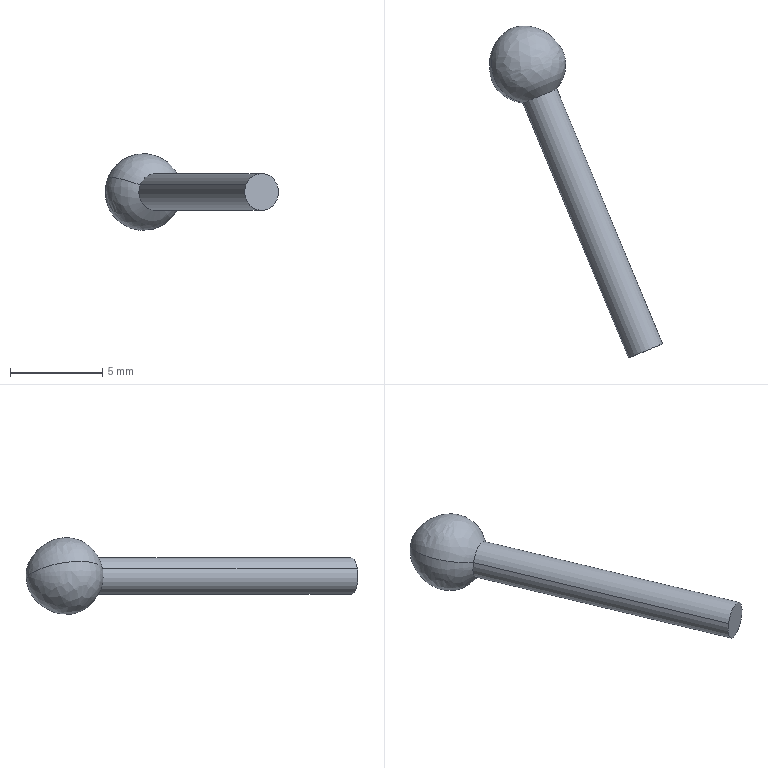Component | SolidWorks | FixedSign-2 | 1 solid | 5 faces | box 9.42 x 18.04 x 4.17 mm | volume 85 mm3 | spline 2 | cylinder 2 | plane 1 | commonest cylinder face diameters 2 x2
STEP:
#1=COLOUR_RGB('',0.7922,0.8196,0.9333);
#2=FILL_AREA_STYLE_COLOUR('',#1);
#3=FILL_AREA_STYLE('',(#2));
#4=SURFACE_STYLE_FILL_AREA(#3);
#5=SURFACE_SIDE_STYLE('',(#4));
#6=SURFACE_STYLE_USAGE(.BOTH.,#5);
#7=PRESENTATION_STYLE_ASSIGNMENT((#6));
#8=CARTESIAN_POINT('',(1.156,0.4229,15.565));
#9=VERTEX_POINT('',#8);
#10=CARTESIAN_POINT('',(1.182,0.264,15.58));
#11=VERTEX_POINT('',#10);
#12=CARTESIAN_POINT('',(1.156,0.4229,15.565));
#13=CARTESIAN_POINT('',(1.095,0.3958,15.592));
#14=CARTESIAN_POINT('',(1.093,0.2788,15.612));
#15=CARTESIAN_POINT('',(1.182,0.264,15.58));
#16=B_SPLINE_CURVE_WITH_KNOTS('',3,(#12,#13,#14,#15),.UNSPECIFIED.,.F.,.F.,(4,4),(0.,1.),.UNSPECIFIED.);
#17=EDGE_CURVE('',#9,#11,#16,.T.);
#18=ORIENTED_EDGE('',*,*,#17,.F.);
#19=CARTESIAN_POINT('',(1.249,0.2919,15.55));
#20=VERTEX_POINT('',#19);
#21=CARTESIAN_POINT('',(1.156,0.4229,15.565));
#22=CARTESIAN_POINT('',(1.217,0.4464,15.537));
#23=CARTESIAN_POINT('',(1.302,0.3653,15.518));
#24=CARTESIAN_POINT('',(1.249,0.2919,15.55));
#25=B_SPLINE_CURVE_WITH_KNOTS('',3,(#21,#22,#23,#24),.UNSPECIFIED.,.F.,.F.,(4,4),(0.,1.),.UNSPECIFIED.);
#26=EDGE_CURVE('',#9,#20,#25,.T.);
#27=ORIENTED_EDGE('',*,*,#26,.T.);
#28=CARTESIAN_POINT('',(1.216,0.278,15.565));
#29=DIRECTION('',(-0.383,0.9237,0.));
#30=DIRECTION('',(-0.8533,-0.3538,0.383));
#31=AXIS2_PLACEMENT_3D('',#28,#29,#30);
#32=CIRCLE('',#31,0.03937);
#33=EDGE_CURVE('',#20,#11,#32,.T.);
#34=ORIENTED_EDGE('',*,*,#33,.T.);
#35=EDGE_LOOP('',(#18,#27,#34));
#36=FACE_OUTER_BOUND('',#35,.T.);
#37=CARTESIAN_POINT('',(1.156,0.4229,15.565));
#38=CARTESIAN_POINT('',(1.156,0.4229,15.565));
#39=CARTESIAN_POINT('',(1.156,0.4229,15.565));
#40=CARTESIAN_POINT('',(1.156,0.4229,15.565));
#41=CARTESIAN_POINT('',(1.217,0.4464,15.537));
#42=CARTESIAN_POINT('',(1.167,0.4254,15.406));
#43=CARTESIAN_POINT('',(1.045,0.3749,15.46));
#44=CARTESIAN_POINT('',(1.095,0.3958,15.592));
#45=CARTESIAN_POINT('',(1.302,0.3653,15.518));
#46=CARTESIAN_POINT('',(1.215,0.3294,15.292));
#47=CARTESIAN_POINT('',(1.007,0.2429,15.386));
#48=CARTESIAN_POINT('',(1.093,0.2788,15.612));
#49=CARTESIAN_POINT('',(1.249,0.2919,15.55));
#50=CARTESIAN_POINT('',(1.221,0.2803,15.477));
#51=CARTESIAN_POINT('',(1.154,0.2525,15.507));
#52=CARTESIAN_POINT('',(1.182,0.264,15.58));
#53=(BOUNDED_SURFACE()B_SPLINE_SURFACE(3,3,((#37,#38,#39,#40),(#41,#42,#43,#44),(#45,#46,#47,#48),(#49,#50,#51,#52)),.UNSPECIFIED.,.F.,.F.,.T.)B_SPLINE_SURFACE_WITH_KNOTS((4,4),(4,4),(0.,1.),(0.,1.),.UNSPECIFIED.)GEOMETRIC_REPRESENTATION_ITEM()RATIONAL_B_SPLINE_SURFACE(((1.,0.3333,0.3333,1.),(1.,0.3333,0.3333,1.),(1.,0.3333,0.3333,1.),(1.,0.3333,0.3333,1.)))REPRESENTATION_ITEM('')SURFACE());
#54=ADVANCED_FACE('',(#36),#53,.T.);
#55=CARTESIAN_POINT('',(1.475,-0.2536,15.55));
#56=VERTEX_POINT('',#55);
#57=CARTESIAN_POINT('',(1.408,-0.2815,15.58));
#58=VERTEX_POINT('',#57);
#59=CARTESIAN_POINT('',(1.442,-0.2675,15.565));
#60=DIRECTION('',(0.383,-0.9237,0.));
#61=DIRECTION('',(0.8533,0.3538,-0.383));
#62=AXIS2_PLACEMENT_3D('',#59,#60,#61);
#63=CIRCLE('',#62,0.03937);
#64=EDGE_CURVE('',#56,#58,#63,.T.);
#65=ORIENTED_EDGE('',*,*,#64,.F.);
#66=CARTESIAN_POINT('',(1.475,-0.2536,15.55));
#67=DIRECTION('',(-0.383,0.9237,0.));
#68=VECTOR('',#67,39.37);
#69=LINE('',#66,#68);
#70=EDGE_CURVE('',#56,#20,#69,.T.);
#71=ORIENTED_EDGE('',*,*,#70,.T.);
#72=CARTESIAN_POINT('',(1.216,0.278,15.565));
#73=DIRECTION('',(-0.383,0.9237,0.));
#74=DIRECTION('',(-0.8533,-0.3538,0.383));
#75=AXIS2_PLACEMENT_3D('',#72,#73,#74);
#76=CIRCLE('',#75,0.03937);
#77=EDGE_CURVE('',#11,#20,#76,.T.);
#78=ORIENTED_EDGE('',*,*,#77,.F.);
#79=CARTESIAN_POINT('',(1.408,-0.2815,15.58));
#80=DIRECTION('',(-0.383,0.9237,0.));
#81=VECTOR('',#80,39.37);
#82=LINE('',#79,#81);
#83=EDGE_CURVE('',#58,#11,#82,.T.);
#84=ORIENTED_EDGE('',*,*,#83,.F.);
#85=EDGE_LOOP('',(#65,#71,#78,#84));
#86=FACE_OUTER_BOUND('',#85,.T.);
#87=CARTESIAN_POINT('',(1.442,-0.2675,15.565));
#88=DIRECTION('',(-0.383,0.9237,0.));
#89=DIRECTION('',(-0.8533,-0.3538,0.383));
#90=AXIS2_PLACEMENT_3D('',#87,#88,#89);
#91=CYLINDRICAL_SURFACE('',#90,0.03937);
#92=ADVANCED_FACE('',(#86),#91,.T.);
#93=ORIENTED_EDGE('',*,*,#70,.F.);
#94=CARTESIAN_POINT('',(1.442,-0.2675,15.565));
#95=DIRECTION('',(0.383,-0.9237,0.));
#96=DIRECTION('',(0.8533,0.3538,-0.383));
#97=AXIS2_PLACEMENT_3D('',#94,#95,#96);
#98=CIRCLE('',#97,0.03937);
#99=EDGE_CURVE('',#58,#56,#98,.T.);
#100=ORIENTED_EDGE('',*,*,#99,.F.);
#101=ORIENTED_EDGE('',*,*,#83,.T.);
#102=ORIENTED_EDGE('',*,*,#33,.F.);
#103=EDGE_LOOP('',(#93,#100,#101,#102));
#104=FACE_OUTER_BOUND('',#103,.T.);
#105=CARTESIAN_POINT('',(1.442,-0.2675,15.565));
#106=DIRECTION('',(-0.383,0.9237,0.));
#107=DIRECTION('',(-0.8533,-0.3538,0.383));
#108=AXIS2_PLACEMENT_3D('',#105,#106,#107);
#109=CYLINDRICAL_SURFACE('',#108,0.03937);
#110=ADVANCED_FACE('',(#104),#109,.T.);
#111=ORIENTED_EDGE('',*,*,#99,.T.);
#112=ORIENTED_EDGE('',*,*,#64,.T.);
#113=EDGE_LOOP('',(#111,#112));
#114=FACE_OUTER_BOUND('',#113,.T.);
#115=CARTESIAN_POINT('',(1.442,-0.2675,15.565));
#116=DIRECTION('',(0.383,-0.9237,-0.));
#117=DIRECTION('',(0.8533,0.3538,-0.383));
#118=AXIS2_PLACEMENT_3D('',#115,#116,#117);
#119=PLANE('',#118);
#120=ADVANCED_FACE('',(#114),#119,.T.);
#121=ORIENTED_EDGE('',*,*,#26,.F.);
#122=ORIENTED_EDGE('',*,*,#17,.T.);
#123=ORIENTED_EDGE('',*,*,#77,.T.);
#124=EDGE_LOOP('',(#121,#122,#123));
#125=FACE_OUTER_BOUND('',#124,.T.);
#126=CARTESIAN_POINT('',(1.156,0.4229,15.565));
#127=CARTESIAN_POINT('',(1.156,0.4229,15.565));
#128=CARTESIAN_POINT('',(1.156,0.4229,15.565));
#129=CARTESIAN_POINT('',(1.156,0.4229,15.565));
#130=CARTESIAN_POINT('',(1.095,0.3958,15.592));
#131=CARTESIAN_POINT('',(1.146,0.4168,15.724));
#132=CARTESIAN_POINT('',(1.268,0.4673,15.669));
#133=CARTESIAN_POINT('',(1.217,0.4464,15.537));
#134=CARTESIAN_POINT('',(1.093,0.2788,15.612));
#135=CARTESIAN_POINT('',(1.18,0.3146,15.837));
#136=CARTESIAN_POINT('',(1.388,0.4011,15.744));
#137=CARTESIAN_POINT('',(1.302,0.3653,15.518));
#138=CARTESIAN_POINT('',(1.182,0.264,15.58));
#139=CARTESIAN_POINT('',(1.21,0.2756,15.653));
#140=CARTESIAN_POINT('',(1.277,0.3035,15.622));
#141=CARTESIAN_POINT('',(1.249,0.2919,15.55));
#142=(BOUNDED_SURFACE()B_SPLINE_SURFACE(3,3,((#126,#127,#128,#129),(#130,#131,#132,#133),(#134,#135,#136,#137),(#138,#139,#140,#141)),.UNSPECIFIED.,.F.,.F.,.T.)B_SPLINE_SURFACE_WITH_KNOTS((4,4),(4,4),(0.,1.),(0.,1.),.UNSPECIFIED.)GEOMETRIC_REPRESENTATION_ITEM()RATIONAL_B_SPLINE_SURFACE(((1.,0.3333,0.3333,1.),(1.,0.3333,0.3333,1.),(1.,0.3333,0.3333,1.),(1.,0.3333,0.3333,1.)))REPRESENTATION_ITEM('')SURFACE());
#143=ADVANCED_FACE('',(#125),#142,.T.);
#144=CLOSED_SHELL('',(#54,#92,#110,#120,#143));
#145=MANIFOLD_SOLID_BREP('',#144);
#146=STYLED_ITEM('',(#7),#145);
#147=PRESENTATION_LAYER_ASSIGNMENT('','',(#146));
#148=(LENGTH_UNIT()NAMED_UNIT(*)SI_UNIT($,.METRE.));
#149=LENGTH_MEASURE_WITH_UNIT(LENGTH_MEASURE(0.0254),#148);
#150=DIMENSIONAL_EXPONENTS(1.,0.,0.,0.,0.,0.,0.);
#151=(CONVERSION_BASED_UNIT('',#149)LENGTH_UNIT()NAMED_UNIT(#150));
#152=UNCERTAINTY_MEASURE_WITH_UNIT(LENGTH_MEASURE(0.00001),#151,'','');
#153=(NAMED_UNIT(*)PLANE_ANGLE_UNIT()SI_UNIT($,.RADIAN.));
#154=(NAMED_UNIT(*)SI_UNIT($,.STERADIAN.)SOLID_ANGLE_UNIT());
#155=(GEOMETRIC_REPRESENTATION_CONTEXT(3)GLOBAL_UNCERTAINTY_ASSIGNED_CONTEXT((#152))GLOBAL_UNIT_ASSIGNED_CONTEXT((#151,#153,#154))REPRESENTATION_CONTEXT('',''));
#156=MECHANICAL_DESIGN_GEOMETRIC_PRESENTATION_REPRESENTATION('',(#146),#155);
#157=CARTESIAN_POINT('',(0.,0.,0.));
#158=DIRECTION('',(0.,0.,1.));
#159=DIRECTION('',(1.,0.,0.));
#160=AXIS2_PLACEMENT_3D('',#157,#158,#159);
#161=(LENGTH_UNIT()NAMED_UNIT(*)SI_UNIT($,.METRE.));
#162=LENGTH_MEASURE_WITH_UNIT(LENGTH_MEASURE(0.0254),#161);
#163=DIMENSIONAL_EXPONENTS(1.,0.,0.,0.,0.,0.,0.);
#164=(CONVERSION_BASED_UNIT('',#162)LENGTH_UNIT()NAMED_UNIT(#163));
#165=UNCERTAINTY_MEASURE_WITH_UNIT(LENGTH_MEASURE(0.00001),#164,'','');
#166=(NAMED_UNIT(*)PLANE_ANGLE_UNIT()SI_UNIT($,.RADIAN.));
#167=(NAMED_UNIT(*)SI_UNIT($,.STERADIAN.)SOLID_ANGLE_UNIT());
#168=(GEOMETRIC_REPRESENTATION_CONTEXT(3)GLOBAL_UNCERTAINTY_ASSIGNED_CONTEXT((#165))GLOBAL_UNIT_ASSIGNED_CONTEXT((#164,#166,#167))REPRESENTATION_CONTEXT('',''));
#169=ADVANCED_BREP_SHAPE_REPRESENTATION('',(#145,#160),#168);